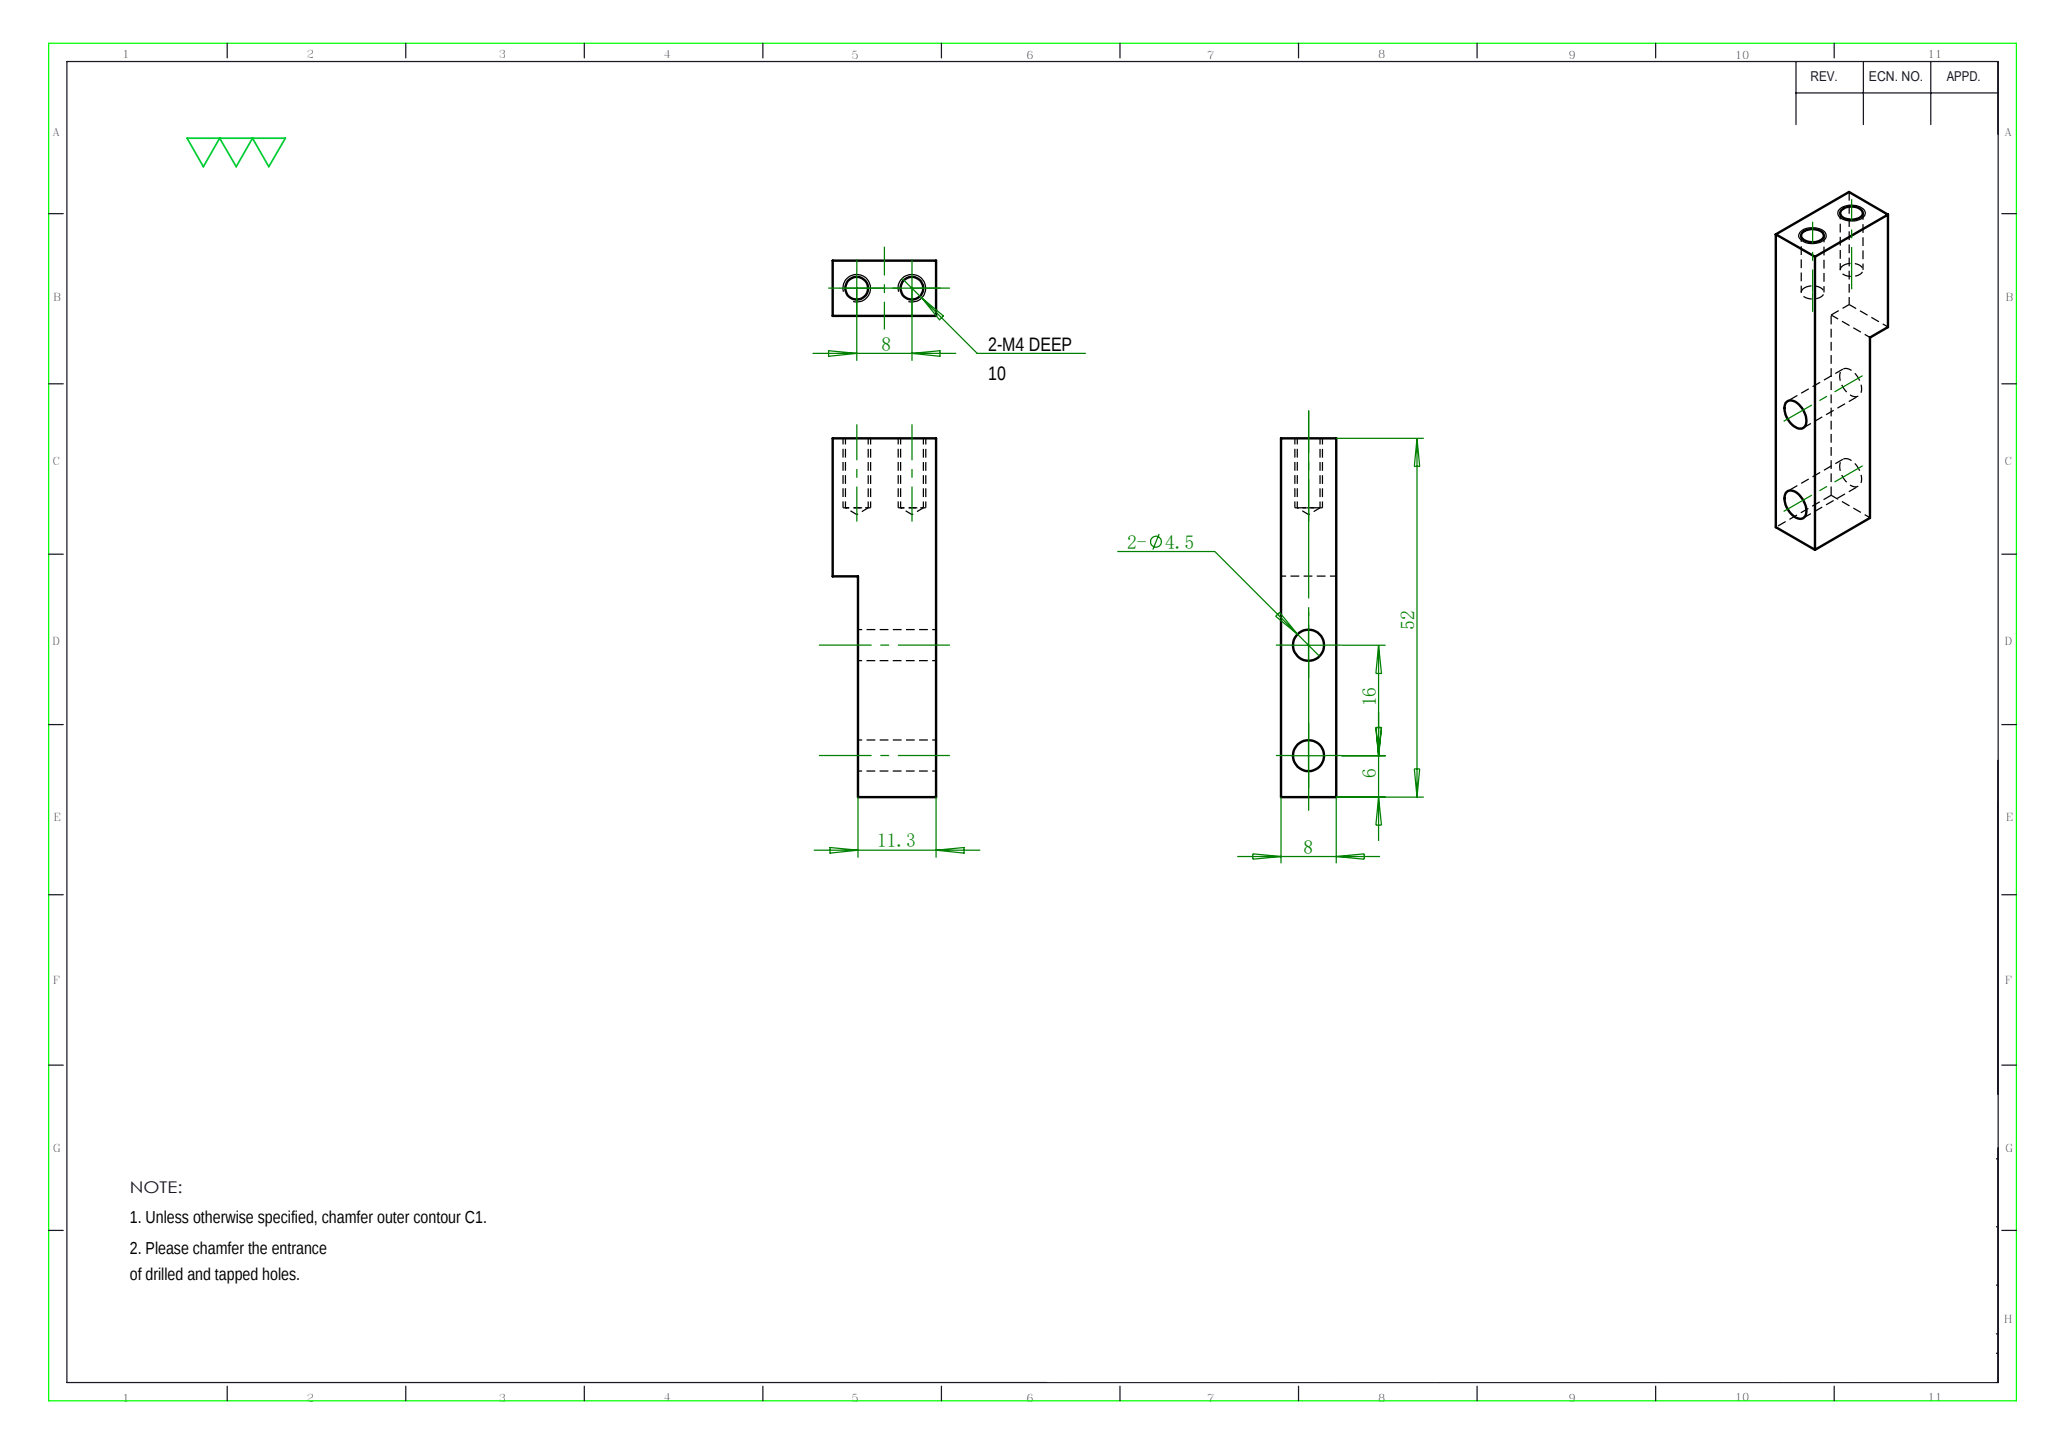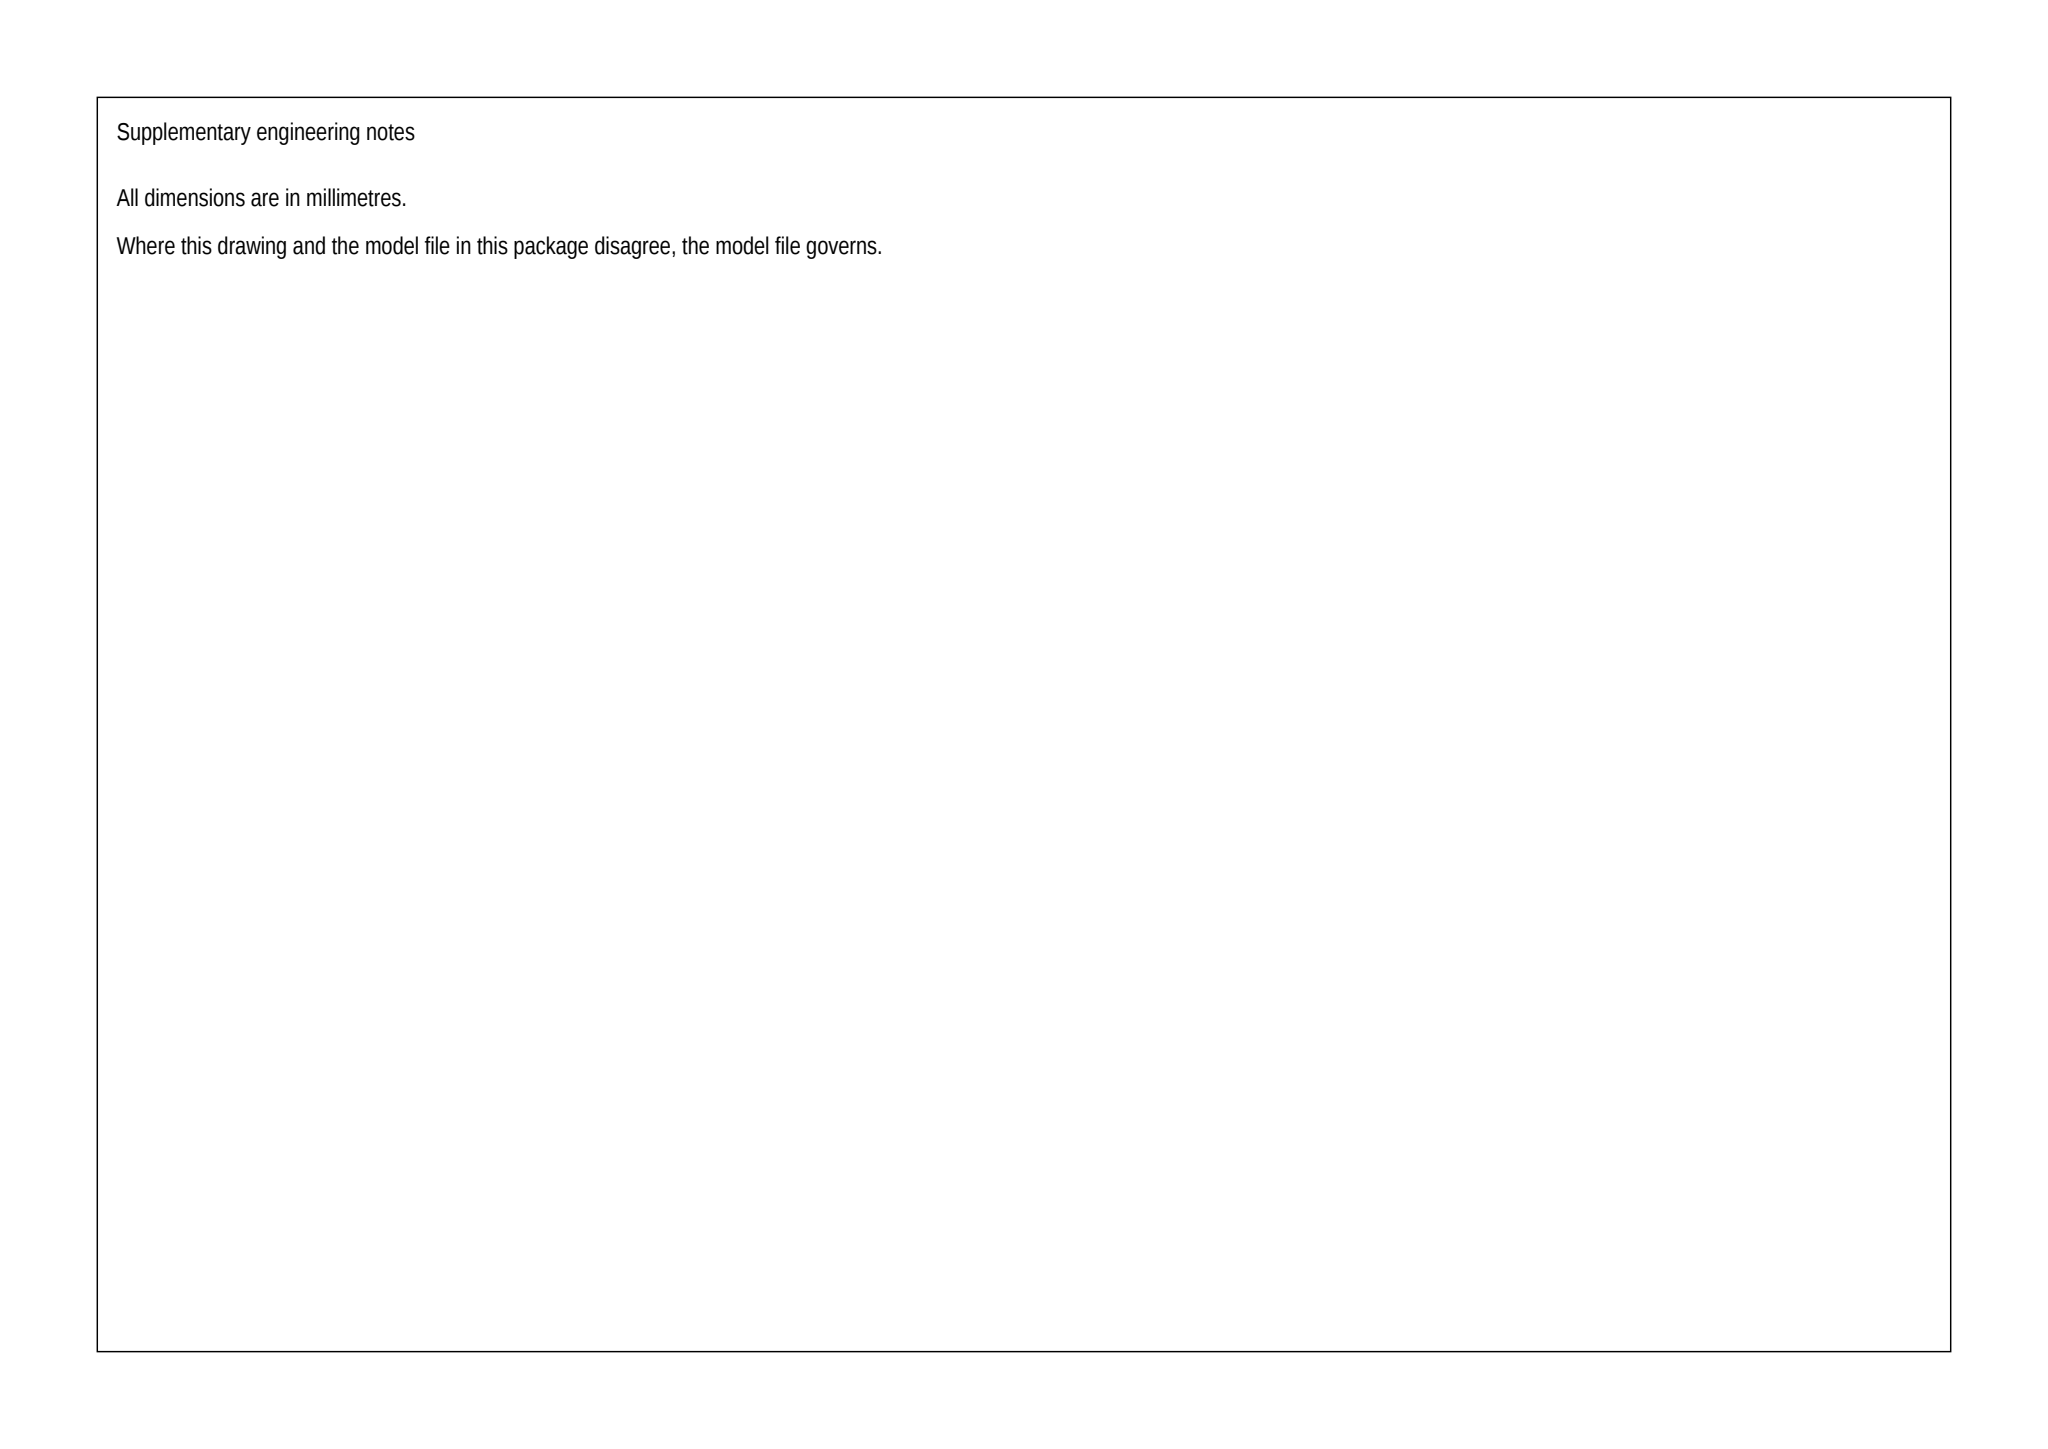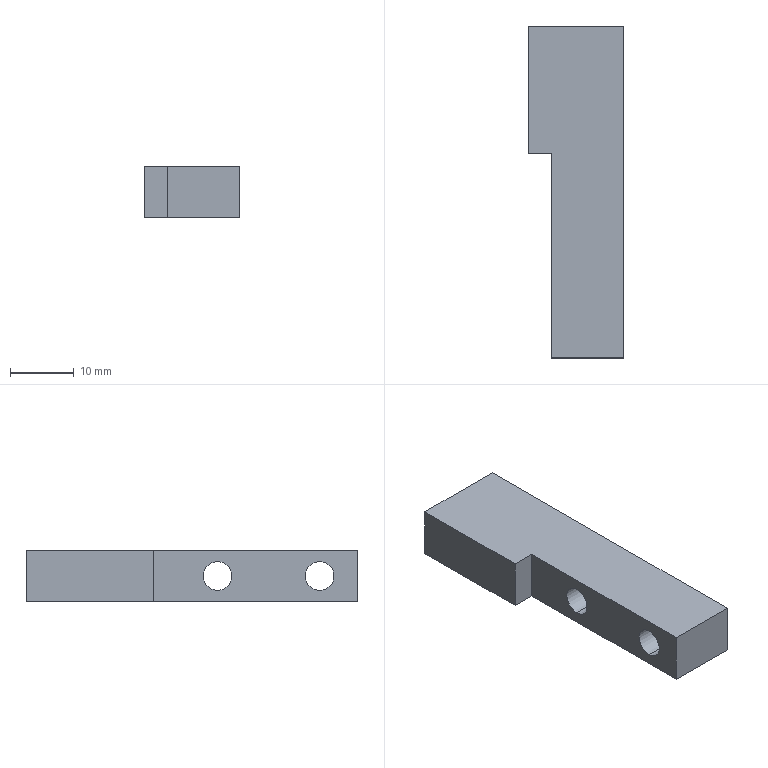Part | SolidWorks | mm | 1 solid | 20 faces | box 15 x 52 x 8 mm | volume 4755 mm3 | cylinder 8 | plane 8 | cone 4 | commonest cylinder face diameters 3.3 x4 4.5 x4
build123d program:
from build123d import *

# Parameters (mm, degrees)
SKETCH1_W                  = 15
SKETCH1_H                  = 52
BOSS_EXTRUDE1_DEPTH        = 8
F_4_5_4_5_DIAMETER_HOLE1_D = 4.5
M4_TAPPED_HOLE1_D          = 3.3
M4_TAPPED_HOLE1_DEPTH      = 10.1
M4_TAPPED_HOLE1_TIP        = 0.9914
SKETCH7_W                  = 3.7
SKETCH7_H                  = 32
CUT_EXTRUDE1_DEPTH         = 29.218


with BuildPart() as part:
    # Sketch1 → Boss-Extrude1 (new body)
    with BuildSketch(Plane.XY):
        Rectangle(SKETCH1_W, SKETCH1_H)
    extrude(amount=BOSS_EXTRUDE1_DEPTH)

    # 4.5 _4.5_ Diameter Hole1 (through all)
    with Locations(Plane.ZY.offset(7.5)):
        with Locations((4, -20), (4, -4)):
            Hole(F_4_5_4_5_DIAMETER_HOLE1_D / 2)

    # M4 Tapped Hole1
    with Locations(Plane(origin=(0, 26, 0), x_dir=(1, 0, 0), z_dir=(0, 1, 0))):
        with Locations((-4, -4), (4, -4)):
            Hole(M4_TAPPED_HOLE1_D / 2, depth=M4_TAPPED_HOLE1_DEPTH)
            with Locations((0, 0, -(M4_TAPPED_HOLE1_DEPTH + M4_TAPPED_HOLE1_TIP / 2))):  # 118° drill point
                Cone(0, M4_TAPPED_HOLE1_D / 2, M4_TAPPED_HOLE1_TIP, mode=Mode.SUBTRACT)

    # Sketch7 → Cut-Extrude1 (cut, through all)
    with BuildSketch(Plane.XY.offset(8)):
        with Locations((-5.65, -10)):
            Rectangle(SKETCH7_W, SKETCH7_H)
    extrude(amount=-CUT_EXTRUDE1_DEPTH, mode=Mode.SUBTRACT)


solid = part.part
STEP:
#1=CARTESIAN_POINT('',(-4.,15.9,2.35));
#2=VERTEX_POINT('',#1);
#3=CARTESIAN_POINT('',(-4.,15.9,5.65));
#4=VERTEX_POINT('',#3);
#5=CARTESIAN_POINT('',(-4.,15.9,4.));
#6=DIRECTION('',(0.,1.,0.));
#7=DIRECTION('',(0.,0.,1.));
#8=AXIS2_PLACEMENT_3D('',#5,#6,#7);
#9=CIRCLE('',#8,1.65);
#10=EDGE_CURVE('',#2,#4,#9,.T.);
#11=ORIENTED_EDGE('',*,*,#10,.F.);
#12=CARTESIAN_POINT('',(-4.,26.,2.35));
#13=VERTEX_POINT('',#12);
#14=CARTESIAN_POINT('',(-4.,26.,2.35));
#15=DIRECTION('',(0.,1.,0.));
#16=VECTOR('',#15,1000.);
#17=LINE('',#14,#16);
#18=EDGE_CURVE('',#2,#13,#17,.T.);
#19=ORIENTED_EDGE('',*,*,#18,.T.);
#20=CARTESIAN_POINT('',(-4.,26.,5.65));
#21=VERTEX_POINT('',#20);
#22=CARTESIAN_POINT('',(-4.,26.,4.));
#23=DIRECTION('',(0.,1.,0.));
#24=DIRECTION('',(0.,0.,1.));
#25=AXIS2_PLACEMENT_3D('',#22,#23,#24);
#26=CIRCLE('',#25,1.65);
#27=EDGE_CURVE('',#13,#21,#26,.T.);
#28=ORIENTED_EDGE('',*,*,#27,.T.);
#29=CARTESIAN_POINT('',(-4.,26.,5.65));
#30=DIRECTION('',(0.,1.,0.));
#31=VECTOR('',#30,1000.);
#32=LINE('',#29,#31);
#33=EDGE_CURVE('',#4,#21,#32,.T.);
#34=ORIENTED_EDGE('',*,*,#33,.F.);
#35=EDGE_LOOP('',(#11,#19,#28,#34));
#36=FACE_OUTER_BOUND('',#35,.T.);
#37=CARTESIAN_POINT('',(-4.,26.,4.));
#38=DIRECTION('',(0.,1.,0.));
#39=DIRECTION('',(0.,0.,1.));
#40=AXIS2_PLACEMENT_3D('',#37,#38,#39);
#41=CYLINDRICAL_SURFACE('',#40,1.65);
#42=ADVANCED_FACE('',(#36),#41,.F.);
#43=CARTESIAN_POINT('',(-4.,14.909,4.));
#44=VERTEX_POINT('',#43);
#45=CARTESIAN_POINT('',(-4.,15.9,5.65));
#46=DIRECTION('',(0.,0.515,0.8572));
#47=VECTOR('',#46,1000.);
#48=LINE('',#45,#47);
#49=EDGE_CURVE('',#44,#4,#48,.T.);
#50=ORIENTED_EDGE('',*,*,#49,.F.);
#51=CARTESIAN_POINT('',(-4.,15.9,2.35));
#52=DIRECTION('',(0.,0.515,-0.8572));
#53=VECTOR('',#52,1000.);
#54=LINE('',#51,#53);
#55=EDGE_CURVE('',#44,#2,#54,.T.);
#56=ORIENTED_EDGE('',*,*,#55,.T.);
#57=ORIENTED_EDGE('',*,*,#10,.T.);
#58=EDGE_LOOP('',(#50,#56,#57));
#59=FACE_OUTER_BOUND('',#58,.T.);
#60=CARTESIAN_POINT('',(-4.,15.9,4.));
#61=DIRECTION('',(0.,1.,0.));
#62=DIRECTION('',(0.,0.,1.));
#63=AXIS2_PLACEMENT_3D('',#60,#61,#62);
#64=CONICAL_SURFACE('',#63,1.65,1.03);
#65=ADVANCED_FACE('',(#59),#64,.F.);
#66=CARTESIAN_POINT('',(4.,15.9,2.35));
#67=VERTEX_POINT('',#66);
#68=CARTESIAN_POINT('',(4.,15.9,5.65));
#69=VERTEX_POINT('',#68);
#70=CARTESIAN_POINT('',(4.,15.9,4.));
#71=DIRECTION('',(0.,1.,0.));
#72=DIRECTION('',(0.,0.,1.));
#73=AXIS2_PLACEMENT_3D('',#70,#71,#72);
#74=CIRCLE('',#73,1.65);
#75=EDGE_CURVE('',#67,#69,#74,.T.);
#76=ORIENTED_EDGE('',*,*,#75,.F.);
#77=CARTESIAN_POINT('',(4.,26.,2.35));
#78=VERTEX_POINT('',#77);
#79=CARTESIAN_POINT('',(4.,26.,2.35));
#80=DIRECTION('',(0.,1.,0.));
#81=VECTOR('',#80,1000.);
#82=LINE('',#79,#81);
#83=EDGE_CURVE('',#67,#78,#82,.T.);
#84=ORIENTED_EDGE('',*,*,#83,.T.);
#85=CARTESIAN_POINT('',(4.,26.,5.65));
#86=VERTEX_POINT('',#85);
#87=CARTESIAN_POINT('',(4.,26.,4.));
#88=DIRECTION('',(0.,1.,0.));
#89=DIRECTION('',(0.,0.,1.));
#90=AXIS2_PLACEMENT_3D('',#87,#88,#89);
#91=CIRCLE('',#90,1.65);
#92=EDGE_CURVE('',#78,#86,#91,.T.);
#93=ORIENTED_EDGE('',*,*,#92,.T.);
#94=CARTESIAN_POINT('',(4.,26.,5.65));
#95=DIRECTION('',(0.,1.,0.));
#96=VECTOR('',#95,1000.);
#97=LINE('',#94,#96);
#98=EDGE_CURVE('',#69,#86,#97,.T.);
#99=ORIENTED_EDGE('',*,*,#98,.F.);
#100=EDGE_LOOP('',(#76,#84,#93,#99));
#101=FACE_OUTER_BOUND('',#100,.T.);
#102=CARTESIAN_POINT('',(4.,26.,4.));
#103=DIRECTION('',(0.,1.,0.));
#104=DIRECTION('',(0.,0.,1.));
#105=AXIS2_PLACEMENT_3D('',#102,#103,#104);
#106=CYLINDRICAL_SURFACE('',#105,1.65);
#107=ADVANCED_FACE('',(#101),#106,.F.);
#108=CARTESIAN_POINT('',(4.,14.909,4.));
#109=VERTEX_POINT('',#108);
#110=CARTESIAN_POINT('',(4.,15.9,5.65));
#111=DIRECTION('',(0.,0.515,0.8572));
#112=VECTOR('',#111,1000.);
#113=LINE('',#110,#112);
#114=EDGE_CURVE('',#109,#69,#113,.T.);
#115=ORIENTED_EDGE('',*,*,#114,.F.);
#116=CARTESIAN_POINT('',(4.,15.9,2.35));
#117=DIRECTION('',(0.,0.515,-0.8572));
#118=VECTOR('',#117,1000.);
#119=LINE('',#116,#118);
#120=EDGE_CURVE('',#109,#67,#119,.T.);
#121=ORIENTED_EDGE('',*,*,#120,.T.);
#122=ORIENTED_EDGE('',*,*,#75,.T.);
#123=EDGE_LOOP('',(#115,#121,#122));
#124=FACE_OUTER_BOUND('',#123,.T.);
#125=CARTESIAN_POINT('',(4.,15.9,4.));
#126=DIRECTION('',(0.,1.,0.));
#127=DIRECTION('',(0.,0.,1.));
#128=AXIS2_PLACEMENT_3D('',#125,#126,#127);
#129=CONICAL_SURFACE('',#128,1.65,1.03);
#130=ADVANCED_FACE('',(#124),#129,.F.);
#131=CARTESIAN_POINT('',(7.5,-20.,1.75));
#132=VERTEX_POINT('',#131);
#133=CARTESIAN_POINT('',(7.5,-20.,6.25));
#134=VERTEX_POINT('',#133);
#135=CARTESIAN_POINT('',(7.5,-20.,4.));
#136=DIRECTION('',(-1.,0.,0.));
#137=DIRECTION('',(0.,0.,1.));
#138=AXIS2_PLACEMENT_3D('',#135,#136,#137);
#139=CIRCLE('',#138,2.25);
#140=EDGE_CURVE('',#132,#134,#139,.T.);
#141=ORIENTED_EDGE('',*,*,#140,.F.);
#142=CARTESIAN_POINT('',(-3.8,-20.,1.75));
#143=VERTEX_POINT('',#142);
#144=CARTESIAN_POINT('',(-7.5,-20.,1.75));
#145=DIRECTION('',(-1.,0.,0.));
#146=VECTOR('',#145,1000.);
#147=LINE('',#144,#146);
#148=EDGE_CURVE('',#132,#143,#147,.T.);
#149=ORIENTED_EDGE('',*,*,#148,.T.);
#150=CARTESIAN_POINT('',(-3.8,-20.,6.25));
#151=VERTEX_POINT('',#150);
#152=CARTESIAN_POINT('',(-3.8,-20.,4.));
#153=DIRECTION('',(-1.,0.,0.));
#154=DIRECTION('',(0.,0.,-1.));
#155=AXIS2_PLACEMENT_3D('',#152,#153,#154);
#156=CIRCLE('',#155,2.25);
#157=EDGE_CURVE('',#143,#151,#156,.T.);
#158=ORIENTED_EDGE('',*,*,#157,.T.);
#159=CARTESIAN_POINT('',(-7.5,-20.,6.25));
#160=DIRECTION('',(-1.,0.,0.));
#161=VECTOR('',#160,1000.);
#162=LINE('',#159,#161);
#163=EDGE_CURVE('',#134,#151,#162,.T.);
#164=ORIENTED_EDGE('',*,*,#163,.F.);
#165=EDGE_LOOP('',(#141,#149,#158,#164));
#166=FACE_OUTER_BOUND('',#165,.T.);
#167=CARTESIAN_POINT('',(-7.5,-20.,4.));
#168=DIRECTION('',(-1.,0.,0.));
#169=DIRECTION('',(0.,0.,1.));
#170=AXIS2_PLACEMENT_3D('',#167,#168,#169);
#171=CYLINDRICAL_SURFACE('',#170,2.25);
#172=ADVANCED_FACE('',(#166),#171,.F.);
#173=CARTESIAN_POINT('',(7.5,-4.,1.75));
#174=VERTEX_POINT('',#173);
#175=CARTESIAN_POINT('',(7.5,-4.,6.25));
#176=VERTEX_POINT('',#175);
#177=CARTESIAN_POINT('',(7.5,-4.,4.));
#178=DIRECTION('',(-1.,0.,0.));
#179=DIRECTION('',(0.,0.,1.));
#180=AXIS2_PLACEMENT_3D('',#177,#178,#179);
#181=CIRCLE('',#180,2.25);
#182=EDGE_CURVE('',#174,#176,#181,.T.);
#183=ORIENTED_EDGE('',*,*,#182,.F.);
#184=CARTESIAN_POINT('',(-3.8,-4.,1.75));
#185=VERTEX_POINT('',#184);
#186=CARTESIAN_POINT('',(-7.5,-4.,1.75));
#187=DIRECTION('',(-1.,0.,0.));
#188=VECTOR('',#187,1000.);
#189=LINE('',#186,#188);
#190=EDGE_CURVE('',#174,#185,#189,.T.);
#191=ORIENTED_EDGE('',*,*,#190,.T.);
#192=CARTESIAN_POINT('',(-3.8,-4.,6.25));
#193=VERTEX_POINT('',#192);
#194=CARTESIAN_POINT('',(-3.8,-4.,4.));
#195=DIRECTION('',(-1.,0.,0.));
#196=DIRECTION('',(0.,0.,-1.));
#197=AXIS2_PLACEMENT_3D('',#194,#195,#196);
#198=CIRCLE('',#197,2.25);
#199=EDGE_CURVE('',#185,#193,#198,.T.);
#200=ORIENTED_EDGE('',*,*,#199,.T.);
#201=CARTESIAN_POINT('',(-7.5,-4.,6.25));
#202=DIRECTION('',(-1.,0.,0.));
#203=VECTOR('',#202,1000.);
#204=LINE('',#201,#203);
#205=EDGE_CURVE('',#176,#193,#204,.T.);
#206=ORIENTED_EDGE('',*,*,#205,.F.);
#207=EDGE_LOOP('',(#183,#191,#200,#206));
#208=FACE_OUTER_BOUND('',#207,.T.);
#209=CARTESIAN_POINT('',(-7.5,-4.,4.));
#210=DIRECTION('',(-1.,0.,0.));
#211=DIRECTION('',(0.,0.,1.));
#212=AXIS2_PLACEMENT_3D('',#209,#210,#211);
#213=CYLINDRICAL_SURFACE('',#212,2.25);
#214=ADVANCED_FACE('',(#208),#213,.F.);
#215=CARTESIAN_POINT('',(7.5,-20.,4.));
#216=DIRECTION('',(-1.,0.,0.));
#217=DIRECTION('',(0.,0.,1.));
#218=AXIS2_PLACEMENT_3D('',#215,#216,#217);
#219=CIRCLE('',#218,2.25);
#220=EDGE_CURVE('',#134,#132,#219,.T.);
#221=ORIENTED_EDGE('',*,*,#220,.T.);
#222=ORIENTED_EDGE('',*,*,#140,.T.);
#223=EDGE_LOOP('',(#221,#222));
#224=FACE_BOUND('',#223,.T.);
#225=CARTESIAN_POINT('',(7.5,-4.,4.));
#226=DIRECTION('',(-1.,0.,0.));
#227=DIRECTION('',(0.,0.,1.));
#228=AXIS2_PLACEMENT_3D('',#225,#226,#227);
#229=CIRCLE('',#228,2.25);
#230=EDGE_CURVE('',#176,#174,#229,.T.);
#231=ORIENTED_EDGE('',*,*,#230,.T.);
#232=ORIENTED_EDGE('',*,*,#182,.T.);
#233=EDGE_LOOP('',(#231,#232));
#234=FACE_BOUND('',#233,.T.);
#235=CARTESIAN_POINT('',(7.5,-26.,0.));
#236=VERTEX_POINT('',#235);
#237=CARTESIAN_POINT('',(7.5,26.,0.));
#238=VERTEX_POINT('',#237);
#239=CARTESIAN_POINT('',(7.5,26.,0.));
#240=DIRECTION('',(-0.,1.,0.));
#241=VECTOR('',#240,1000.);
#242=LINE('',#239,#241);
#243=EDGE_CURVE('',#236,#238,#242,.T.);
#244=ORIENTED_EDGE('',*,*,#243,.T.);
#245=CARTESIAN_POINT('',(7.5,26.,8.));
#246=VERTEX_POINT('',#245);
#247=CARTESIAN_POINT('',(7.5,26.,8.));
#248=DIRECTION('',(0.,0.,-1.));
#249=VECTOR('',#248,1000.);
#250=LINE('',#247,#249);
#251=EDGE_CURVE('',#246,#238,#250,.T.);
#252=ORIENTED_EDGE('',*,*,#251,.F.);
#253=CARTESIAN_POINT('',(7.5,-26.,8.));
#254=VERTEX_POINT('',#253);
#255=CARTESIAN_POINT('',(7.5,26.,8.));
#256=DIRECTION('',(-0.,1.,0.));
#257=VECTOR('',#256,1000.);
#258=LINE('',#255,#257);
#259=EDGE_CURVE('',#254,#246,#258,.T.);
#260=ORIENTED_EDGE('',*,*,#259,.F.);
#261=CARTESIAN_POINT('',(7.5,-26.,8.));
#262=DIRECTION('',(0.,0.,-1.));
#263=VECTOR('',#262,1000.);
#264=LINE('',#261,#263);
#265=EDGE_CURVE('',#254,#236,#264,.T.);
#266=ORIENTED_EDGE('',*,*,#265,.T.);
#267=EDGE_LOOP('',(#244,#252,#260,#266));
#268=FACE_OUTER_BOUND('',#267,.T.);
#269=CARTESIAN_POINT('',(7.5,26.,8.));
#270=DIRECTION('',(-1.,-0.,0.));
#271=DIRECTION('',(0.,-1.,0.));
#272=AXIS2_PLACEMENT_3D('',#269,#270,#271);
#273=PLANE('',#272);
#274=ADVANCED_FACE('',(#224,#234,#268),#273,.F.);
#275=CARTESIAN_POINT('',(-4.,26.,4.));
#276=DIRECTION('',(0.,1.,0.));
#277=DIRECTION('',(0.,0.,1.));
#278=AXIS2_PLACEMENT_3D('',#275,#276,#277);
#279=CIRCLE('',#278,1.65);
#280=EDGE_CURVE('',#21,#13,#279,.T.);
#281=ORIENTED_EDGE('',*,*,#280,.F.);
#282=ORIENTED_EDGE('',*,*,#27,.F.);
#283=EDGE_LOOP('',(#281,#282));
#284=FACE_BOUND('',#283,.T.);
#285=CARTESIAN_POINT('',(4.,26.,4.));
#286=DIRECTION('',(0.,1.,0.));
#287=DIRECTION('',(0.,0.,1.));
#288=AXIS2_PLACEMENT_3D('',#285,#286,#287);
#289=CIRCLE('',#288,1.65);
#290=EDGE_CURVE('',#86,#78,#289,.T.);
#291=ORIENTED_EDGE('',*,*,#290,.F.);
#292=ORIENTED_EDGE('',*,*,#92,.F.);
#293=EDGE_LOOP('',(#291,#292));
#294=FACE_BOUND('',#293,.T.);
#295=CARTESIAN_POINT('',(-7.5,26.,0.));
#296=VERTEX_POINT('',#295);
#297=CARTESIAN_POINT('',(-7.5,26.,0.));
#298=DIRECTION('',(-1.,0.,0.));
#299=VECTOR('',#298,1000.);
#300=LINE('',#297,#299);
#301=EDGE_CURVE('',#238,#296,#300,.T.);
#302=ORIENTED_EDGE('',*,*,#301,.T.);
#303=CARTESIAN_POINT('',(-7.5,26.,8.));
#304=VERTEX_POINT('',#303);
#305=CARTESIAN_POINT('',(-7.5,26.,8.));
#306=DIRECTION('',(0.,0.,-1.));
#307=VECTOR('',#306,1000.);
#308=LINE('',#305,#307);
#309=EDGE_CURVE('',#304,#296,#308,.T.);
#310=ORIENTED_EDGE('',*,*,#309,.F.);
#311=CARTESIAN_POINT('',(-7.5,26.,8.));
#312=DIRECTION('',(-1.,0.,0.));
#313=VECTOR('',#312,1000.);
#314=LINE('',#311,#313);
#315=EDGE_CURVE('',#246,#304,#314,.T.);
#316=ORIENTED_EDGE('',*,*,#315,.F.);
#317=ORIENTED_EDGE('',*,*,#251,.T.);
#318=EDGE_LOOP('',(#302,#310,#316,#317));
#319=FACE_OUTER_BOUND('',#318,.T.);
#320=CARTESIAN_POINT('',(-7.5,26.,8.));
#321=DIRECTION('',(0.,-1.,0.));
#322=DIRECTION('',(0.,0.,-1.));
#323=AXIS2_PLACEMENT_3D('',#320,#321,#322);
#324=PLANE('',#323);
#325=ADVANCED_FACE('',(#284,#294,#319),#324,.F.);
#326=CARTESIAN_POINT('',(-7.5,6.,0.));
#327=VERTEX_POINT('',#326);
#328=CARTESIAN_POINT('',(-7.5,26.,0.));
#329=DIRECTION('',(0.,-1.,0.));
#330=VECTOR('',#329,1000.);
#331=LINE('',#328,#330);
#332=EDGE_CURVE('',#296,#327,#331,.T.);
#333=ORIENTED_EDGE('',*,*,#332,.T.);
#334=CARTESIAN_POINT('',(-7.5,6.,8.));
#335=VERTEX_POINT('',#334);
#336=CARTESIAN_POINT('',(-7.5,6.,0.));
#337=DIRECTION('',(0.,0.,1.));
#338=VECTOR('',#337,1000.);
#339=LINE('',#336,#338);
#340=EDGE_CURVE('',#327,#335,#339,.T.);
#341=ORIENTED_EDGE('',*,*,#340,.T.);
#342=CARTESIAN_POINT('',(-7.5,26.,8.));
#343=DIRECTION('',(0.,-1.,0.));
#344=VECTOR('',#343,1000.);
#345=LINE('',#342,#344);
#346=EDGE_CURVE('',#304,#335,#345,.T.);
#347=ORIENTED_EDGE('',*,*,#346,.F.);
#348=ORIENTED_EDGE('',*,*,#309,.T.);
#349=EDGE_LOOP('',(#333,#341,#347,#348));
#350=FACE_OUTER_BOUND('',#349,.T.);
#351=CARTESIAN_POINT('',(-7.5,26.,8.));
#352=DIRECTION('',(1.,0.,0.));
#353=DIRECTION('',(-0.,1.,0.));
#354=AXIS2_PLACEMENT_3D('',#351,#352,#353);
#355=PLANE('',#354);
#356=ADVANCED_FACE('',(#350),#355,.F.);
#357=CARTESIAN_POINT('',(-3.8,-26.,8.));
#358=VERTEX_POINT('',#357);
#359=CARTESIAN_POINT('',(-7.5,-26.,8.));
#360=DIRECTION('',(1.,0.,0.));
#361=VECTOR('',#360,1000.);
#362=LINE('',#359,#361);
#363=EDGE_CURVE('',#358,#254,#362,.T.);
#364=ORIENTED_EDGE('',*,*,#363,.F.);
#365=CARTESIAN_POINT('',(-3.8,-26.,0.));
#366=VERTEX_POINT('',#365);
#367=CARTESIAN_POINT('',(-3.8,-26.,0.));
#368=DIRECTION('',(0.,0.,1.));
#369=VECTOR('',#368,1000.);
#370=LINE('',#367,#369);
#371=EDGE_CURVE('',#366,#358,#370,.T.);
#372=ORIENTED_EDGE('',*,*,#371,.F.);
#373=CARTESIAN_POINT('',(-7.5,-26.,0.));
#374=DIRECTION('',(1.,0.,0.));
#375=VECTOR('',#374,1000.);
#376=LINE('',#373,#375);
#377=EDGE_CURVE('',#366,#236,#376,.T.);
#378=ORIENTED_EDGE('',*,*,#377,.T.);
#379=ORIENTED_EDGE('',*,*,#265,.F.);
#380=EDGE_LOOP('',(#364,#372,#378,#379));
#381=FACE_OUTER_BOUND('',#380,.T.);
#382=CARTESIAN_POINT('',(-7.5,-26.,8.));
#383=DIRECTION('',(0.,1.,0.));
#384=DIRECTION('',(0.,0.,1.));
#385=AXIS2_PLACEMENT_3D('',#382,#383,#384);
#386=PLANE('',#385);
#387=ADVANCED_FACE('',(#381),#386,.F.);
#388=CARTESIAN_POINT('',(-3.8,6.,8.));
#389=VERTEX_POINT('',#388);
#390=CARTESIAN_POINT('',(-7.5,6.,8.));
#391=DIRECTION('',(-1.,0.,0.));
#392=VECTOR('',#391,1000.);
#393=LINE('',#390,#392);
#394=EDGE_CURVE('',#389,#335,#393,.T.);
#395=ORIENTED_EDGE('',*,*,#394,.F.);
#396=CARTESIAN_POINT('',(-3.8,-26.,8.));
#397=DIRECTION('',(0.,1.,0.));
#398=VECTOR('',#397,1000.);
#399=LINE('',#396,#398);
#400=EDGE_CURVE('',#358,#389,#399,.T.);
#401=ORIENTED_EDGE('',*,*,#400,.F.);
#402=ORIENTED_EDGE('',*,*,#363,.T.);
#403=ORIENTED_EDGE('',*,*,#259,.T.);
#404=ORIENTED_EDGE('',*,*,#315,.T.);
#405=ORIENTED_EDGE('',*,*,#346,.T.);
#406=EDGE_LOOP('',(#395,#401,#402,#403,#404,#405));
#407=FACE_OUTER_BOUND('',#406,.T.);
#408=CARTESIAN_POINT('',(0.,0.,8.));
#409=DIRECTION('',(0.,0.,1.));
#410=DIRECTION('',(1.,0.,0.));
#411=AXIS2_PLACEMENT_3D('',#408,#409,#410);
#412=PLANE('',#411);
#413=ADVANCED_FACE('',(#407),#412,.T.);
#414=CARTESIAN_POINT('',(-3.8,6.,0.));
#415=VERTEX_POINT('',#414);
#416=CARTESIAN_POINT('',(-3.8,-26.,0.));
#417=DIRECTION('',(0.,1.,0.));
#418=VECTOR('',#417,1000.);
#419=LINE('',#416,#418);
#420=EDGE_CURVE('',#366,#415,#419,.T.);
#421=ORIENTED_EDGE('',*,*,#420,.T.);
#422=CARTESIAN_POINT('',(-7.5,6.,0.));
#423=DIRECTION('',(-1.,0.,0.));
#424=VECTOR('',#423,1000.);
#425=LINE('',#422,#424);
#426=EDGE_CURVE('',#415,#327,#425,.T.);
#427=ORIENTED_EDGE('',*,*,#426,.T.);
#428=ORIENTED_EDGE('',*,*,#332,.F.);
#429=ORIENTED_EDGE('',*,*,#301,.F.);
#430=ORIENTED_EDGE('',*,*,#243,.F.);
#431=ORIENTED_EDGE('',*,*,#377,.F.);
#432=EDGE_LOOP('',(#421,#427,#428,#429,#430,#431));
#433=FACE_OUTER_BOUND('',#432,.T.);
#434=CARTESIAN_POINT('',(0.,0.,0.));
#435=DIRECTION('',(0.,0.,1.));
#436=DIRECTION('',(1.,0.,0.));
#437=AXIS2_PLACEMENT_3D('',#434,#435,#436);
#438=PLANE('',#437);
#439=ADVANCED_FACE('',(#433),#438,.F.);
#440=ORIENTED_EDGE('',*,*,#190,.F.);
#441=ORIENTED_EDGE('',*,*,#230,.F.);
#442=ORIENTED_EDGE('',*,*,#205,.T.);
#443=CARTESIAN_POINT('',(-3.8,-4.,4.));
#444=DIRECTION('',(-1.,0.,0.));
#445=DIRECTION('',(0.,0.,-1.));
#446=AXIS2_PLACEMENT_3D('',#443,#444,#445);
#447=CIRCLE('',#446,2.25);
#448=EDGE_CURVE('',#193,#185,#447,.T.);
#449=ORIENTED_EDGE('',*,*,#448,.T.);
#450=EDGE_LOOP('',(#440,#441,#442,#449));
#451=FACE_OUTER_BOUND('',#450,.T.);
#452=CARTESIAN_POINT('',(-7.5,-4.,4.));
#453=DIRECTION('',(-1.,0.,0.));
#454=DIRECTION('',(0.,0.,1.));
#455=AXIS2_PLACEMENT_3D('',#452,#453,#454);
#456=CYLINDRICAL_SURFACE('',#455,2.25);
#457=ADVANCED_FACE('',(#451),#456,.F.);
#458=ORIENTED_EDGE('',*,*,#148,.F.);
#459=ORIENTED_EDGE('',*,*,#220,.F.);
#460=ORIENTED_EDGE('',*,*,#163,.T.);
#461=CARTESIAN_POINT('',(-3.8,-20.,4.));
#462=DIRECTION('',(-1.,0.,0.));
#463=DIRECTION('',(0.,0.,-1.));
#464=AXIS2_PLACEMENT_3D('',#461,#462,#463);
#465=CIRCLE('',#464,2.25);
#466=EDGE_CURVE('',#151,#143,#465,.T.);
#467=ORIENTED_EDGE('',*,*,#466,.T.);
#468=EDGE_LOOP('',(#458,#459,#460,#467));
#469=FACE_OUTER_BOUND('',#468,.T.);
#470=CARTESIAN_POINT('',(-7.5,-20.,4.));
#471=DIRECTION('',(-1.,0.,0.));
#472=DIRECTION('',(0.,0.,1.));
#473=AXIS2_PLACEMENT_3D('',#470,#471,#472);
#474=CYLINDRICAL_SURFACE('',#473,2.25);
#475=ADVANCED_FACE('',(#469),#474,.F.);
#476=ORIENTED_EDGE('',*,*,#120,.F.);
#477=ORIENTED_EDGE('',*,*,#114,.T.);
#478=CARTESIAN_POINT('',(4.,15.9,4.));
#479=DIRECTION('',(0.,1.,0.));
#480=DIRECTION('',(0.,0.,1.));
#481=AXIS2_PLACEMENT_3D('',#478,#479,#480);
#482=CIRCLE('',#481,1.65);
#483=EDGE_CURVE('',#69,#67,#482,.T.);
#484=ORIENTED_EDGE('',*,*,#483,.T.);
#485=EDGE_LOOP('',(#476,#477,#484));
#486=FACE_OUTER_BOUND('',#485,.T.);
#487=CARTESIAN_POINT('',(4.,15.9,4.));
#488=DIRECTION('',(0.,1.,0.));
#489=DIRECTION('',(0.,0.,1.));
#490=AXIS2_PLACEMENT_3D('',#487,#488,#489);
#491=CONICAL_SURFACE('',#490,1.65,1.03);
#492=ADVANCED_FACE('',(#486),#491,.F.);
#493=ORIENTED_EDGE('',*,*,#83,.F.);
#494=ORIENTED_EDGE('',*,*,#483,.F.);
#495=ORIENTED_EDGE('',*,*,#98,.T.);
#496=ORIENTED_EDGE('',*,*,#290,.T.);
#497=EDGE_LOOP('',(#493,#494,#495,#496));
#498=FACE_OUTER_BOUND('',#497,.T.);
#499=CARTESIAN_POINT('',(4.,26.,4.));
#500=DIRECTION('',(0.,1.,0.));
#501=DIRECTION('',(0.,0.,1.));
#502=AXIS2_PLACEMENT_3D('',#499,#500,#501);
#503=CYLINDRICAL_SURFACE('',#502,1.65);
#504=ADVANCED_FACE('',(#498),#503,.F.);
#505=ORIENTED_EDGE('',*,*,#55,.F.);
#506=ORIENTED_EDGE('',*,*,#49,.T.);
#507=CARTESIAN_POINT('',(-4.,15.9,4.));
#508=DIRECTION('',(0.,1.,0.));
#509=DIRECTION('',(0.,0.,1.));
#510=AXIS2_PLACEMENT_3D('',#507,#508,#509);
#511=CIRCLE('',#510,1.65);
#512=EDGE_CURVE('',#4,#2,#511,.T.);
#513=ORIENTED_EDGE('',*,*,#512,.T.);
#514=EDGE_LOOP('',(#505,#506,#513));
#515=FACE_OUTER_BOUND('',#514,.T.);
#516=CARTESIAN_POINT('',(-4.,15.9,4.));
#517=DIRECTION('',(0.,1.,0.));
#518=DIRECTION('',(0.,0.,1.));
#519=AXIS2_PLACEMENT_3D('',#516,#517,#518);
#520=CONICAL_SURFACE('',#519,1.65,1.03);
#521=ADVANCED_FACE('',(#515),#520,.F.);
#522=ORIENTED_EDGE('',*,*,#18,.F.);
#523=ORIENTED_EDGE('',*,*,#512,.F.);
#524=ORIENTED_EDGE('',*,*,#33,.T.);
#525=ORIENTED_EDGE('',*,*,#280,.T.);
#526=EDGE_LOOP('',(#522,#523,#524,#525));
#527=FACE_OUTER_BOUND('',#526,.T.);
#528=CARTESIAN_POINT('',(-4.,26.,4.));
#529=DIRECTION('',(0.,1.,0.));
#530=DIRECTION('',(0.,0.,1.));
#531=AXIS2_PLACEMENT_3D('',#528,#529,#530);
#532=CYLINDRICAL_SURFACE('',#531,1.65);
#533=ADVANCED_FACE('',(#527),#532,.F.);
#534=ORIENTED_EDGE('',*,*,#466,.F.);
#535=ORIENTED_EDGE('',*,*,#157,.F.);
#536=EDGE_LOOP('',(#534,#535));
#537=FACE_BOUND('',#536,.T.);
#538=ORIENTED_EDGE('',*,*,#400,.T.);
#539=CARTESIAN_POINT('',(-3.8,6.,0.));
#540=DIRECTION('',(0.,0.,1.));
#541=VECTOR('',#540,1000.);
#542=LINE('',#539,#541);
#543=EDGE_CURVE('',#415,#389,#542,.T.);
#544=ORIENTED_EDGE('',*,*,#543,.F.);
#545=ORIENTED_EDGE('',*,*,#420,.F.);
#546=ORIENTED_EDGE('',*,*,#371,.T.);
#547=EDGE_LOOP('',(#538,#544,#545,#546));
#548=FACE_OUTER_BOUND('',#547,.T.);
#549=ORIENTED_EDGE('',*,*,#448,.F.);
#550=ORIENTED_EDGE('',*,*,#199,.F.);
#551=EDGE_LOOP('',(#549,#550));
#552=FACE_BOUND('',#551,.T.);
#553=CARTESIAN_POINT('',(-3.8,-26.,0.));
#554=DIRECTION('',(1.,0.,0.));
#555=DIRECTION('',(0.,0.,-1.));
#556=AXIS2_PLACEMENT_3D('',#553,#554,#555);
#557=PLANE('',#556);
#558=ADVANCED_FACE('',(#537,#548,#552),#557,.F.);
#559=ORIENTED_EDGE('',*,*,#394,.T.);
#560=ORIENTED_EDGE('',*,*,#340,.F.);
#561=ORIENTED_EDGE('',*,*,#426,.F.);
#562=ORIENTED_EDGE('',*,*,#543,.T.);
#563=EDGE_LOOP('',(#559,#560,#561,#562));
#564=FACE_OUTER_BOUND('',#563,.T.);
#565=CARTESIAN_POINT('',(-7.5,6.,0.));
#566=DIRECTION('',(0.,1.,0.));
#567=DIRECTION('',(0.,0.,1.));
#568=AXIS2_PLACEMENT_3D('',#565,#566,#567);
#569=PLANE('',#568);
#570=ADVANCED_FACE('',(#564),#569,.F.);
#571=CLOSED_SHELL('',(#42,#65,#107,#130,#172,#214,#274,#325,#356,#387,#413,#439,#457,#475,#492,#504,#521,#533,#558,#570));
#572=MANIFOLD_SOLID_BREP('',#571);
#573=CARTESIAN_POINT('',(0.,0.,0.));
#574=DIRECTION('',(0.,0.,1.));
#575=DIRECTION('',(1.,0.,0.));
#576=AXIS2_PLACEMENT_3D('',#573,#574,#575);
#577=(LENGTH_UNIT()NAMED_UNIT(*)SI_UNIT(.MILLI.,.METRE.));
#578=UNCERTAINTY_MEASURE_WITH_UNIT(LENGTH_MEASURE(0.00001),#577,'','');
#579=(NAMED_UNIT(*)PLANE_ANGLE_UNIT()SI_UNIT($,.RADIAN.));
#580=(NAMED_UNIT(*)SI_UNIT($,.STERADIAN.)SOLID_ANGLE_UNIT());
#581=(GEOMETRIC_REPRESENTATION_CONTEXT(3)GLOBAL_UNCERTAINTY_ASSIGNED_CONTEXT((#578))GLOBAL_UNIT_ASSIGNED_CONTEXT((#577,#579,#580))REPRESENTATION_CONTEXT('',''));
#582=ADVANCED_BREP_SHAPE_REPRESENTATION('',(#572,#576),#581);